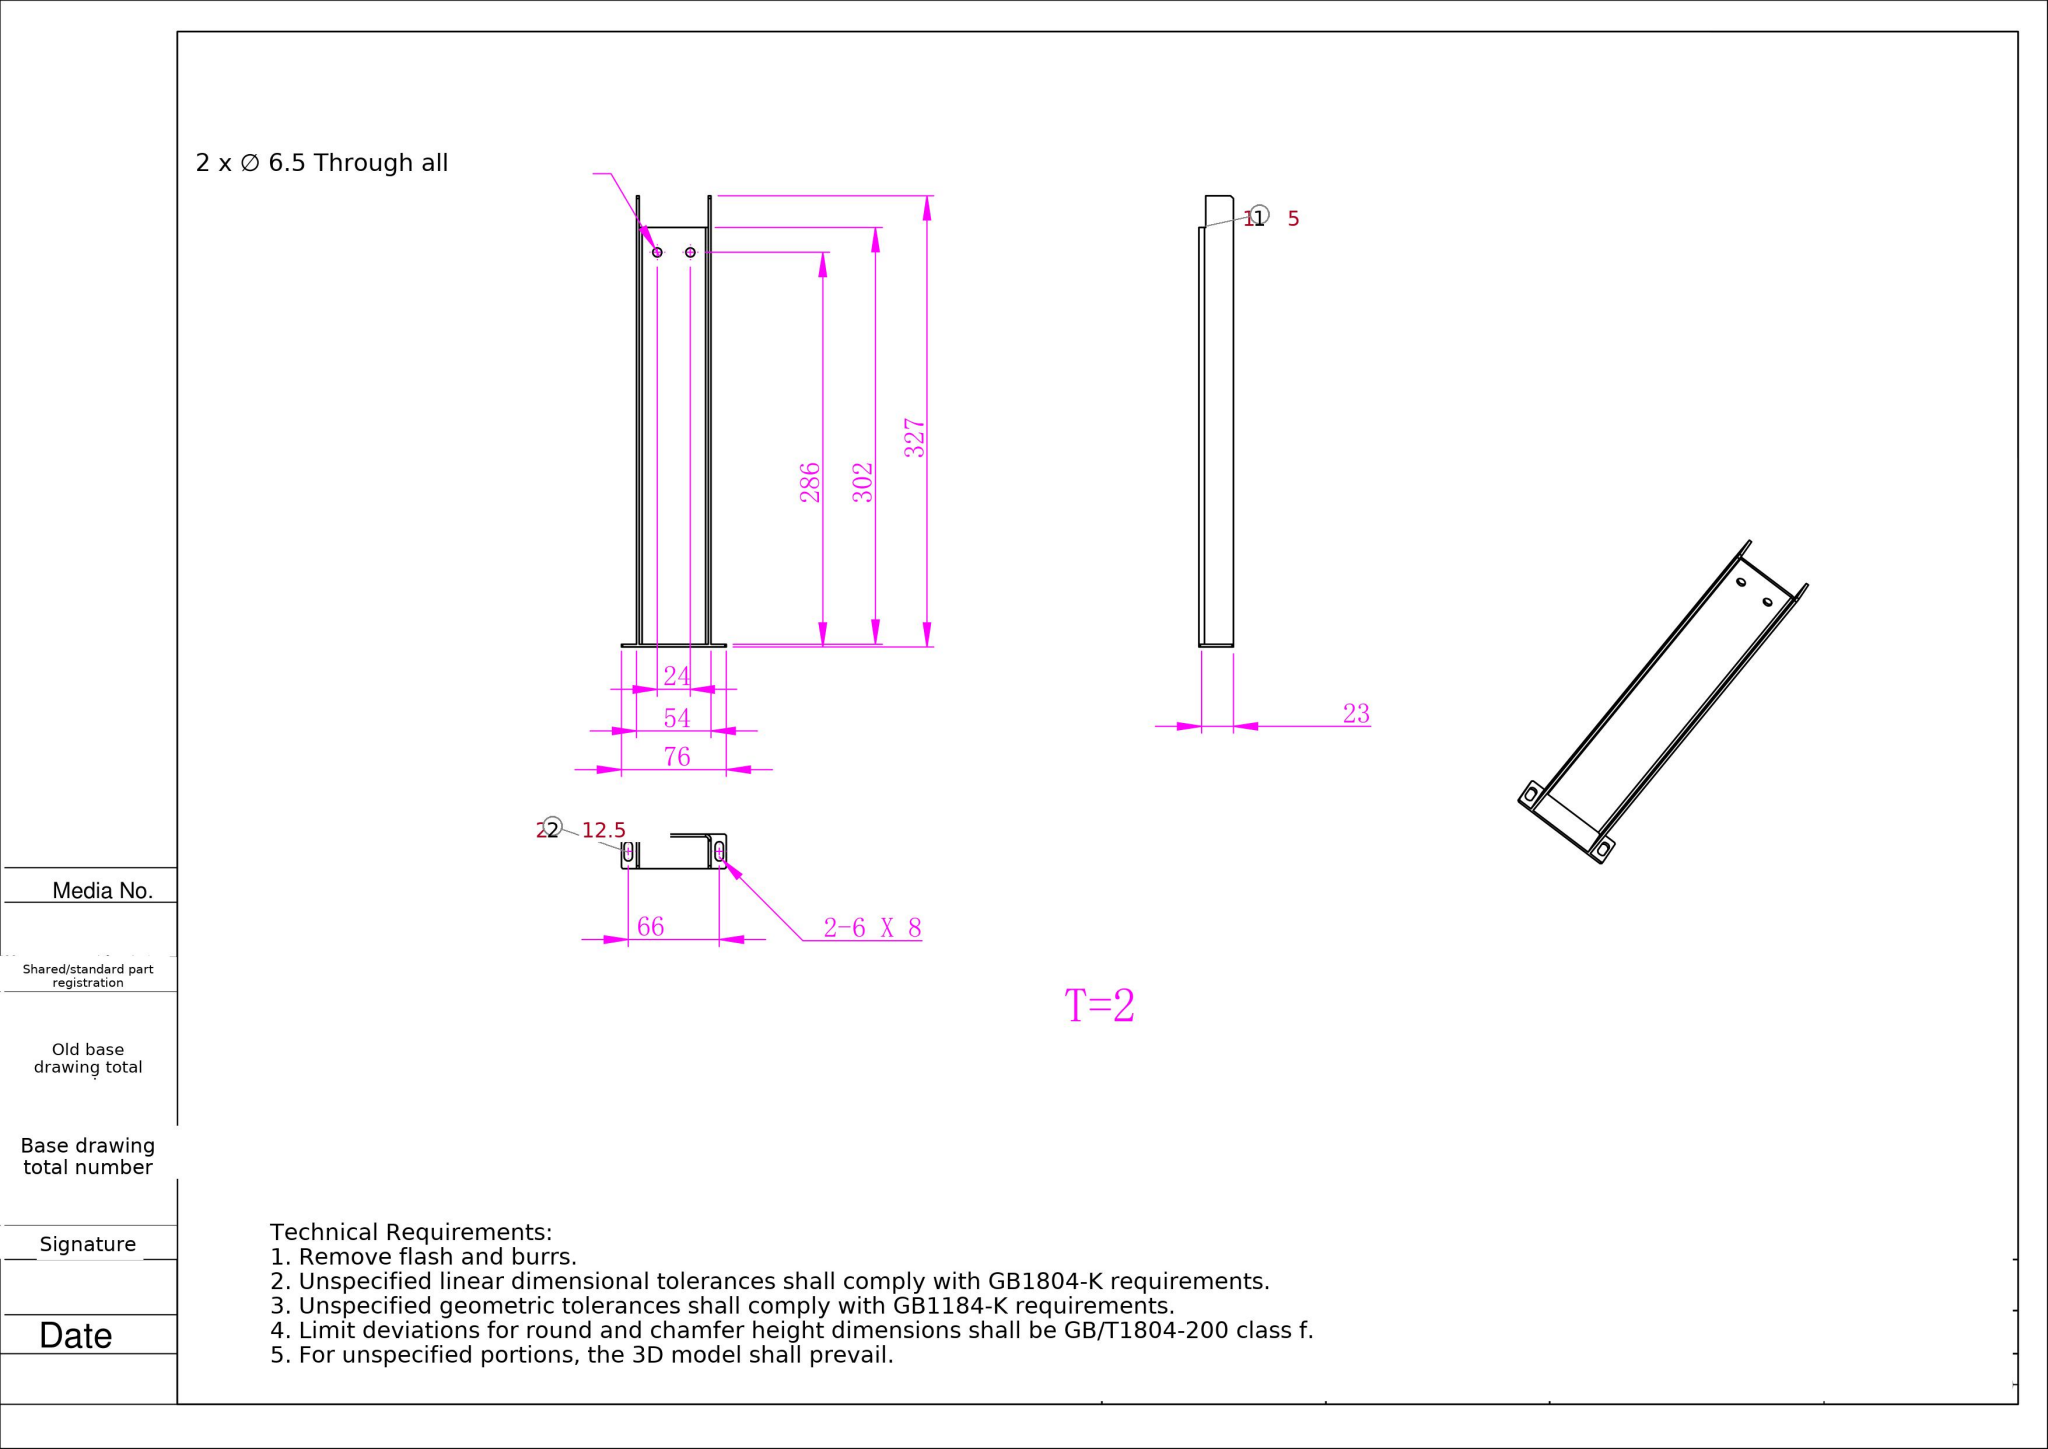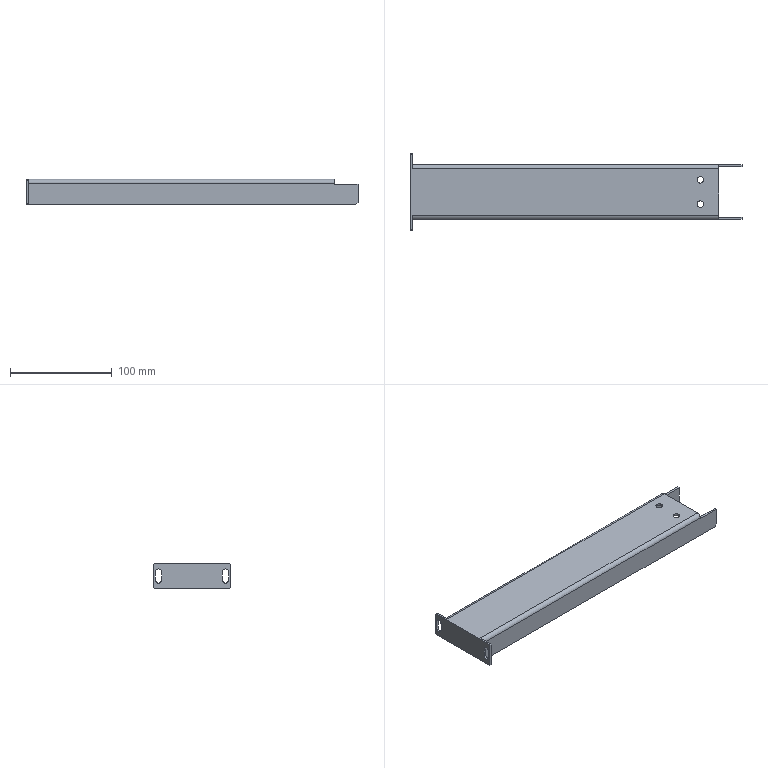Part | SolidWorks | mm | 1 solid | 46 faces | box 327 x 76 x 25 mm | volume 64035 mm3 | plane 32 | cylinder 14 | commonest cylinder face diameters 6 x6 6.5 x4 8 x2 4 x2